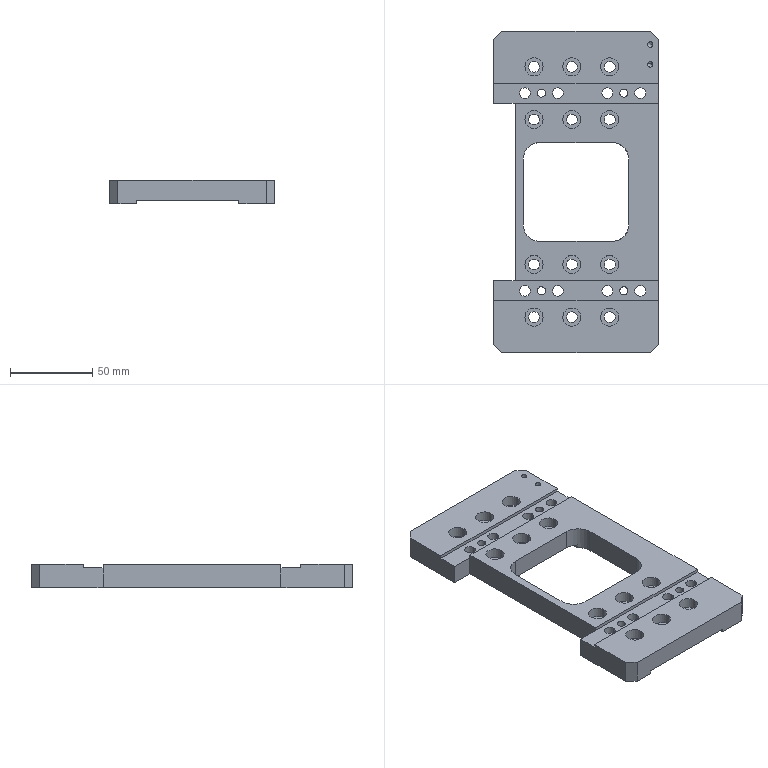Component | SolidWorks | 17081801-804-001A-1 | 1 solid | 155 faces | box 100 x 195 x 14 mm | volume 162308 mm3 | cylinder 96 | plane 55 | cone 4 | commonest cylinder face diameters 11 x40 6.6 x40 5 x8 3.3 x4 20 x4 | material AL6061
build123d program:
from build123d import *

# Parameters (mm, degrees)
SKETCH1_W                                       = 195
SKETCH1_H                                       = 100
BOSS_EXTRUDE1_DEPTH                             = 7
M6_HEX_SOCKET_HEAD_CAP_SCREW_CBORE1_D           = 6.6
M6_HEX_SOCKET_HEAD_CAP_SCREW_CBORE1_CBORE_D     = 11
M6_HEX_SOCKET_HEAD_CAP_SCREW_CBORE1_CBORE_DEPTH = 6.4
LPATTERN1_COUNT                                 = 2
LPATTERN1_PITCH                                 = 120
M6_HEX_SOCKET_HEAD_CAP_SCREW_CBORE2_D           = 6.6
M6_HEX_SOCKET_HEAD_CAP_SCREW_CBORE2_DEPTH       = 56
M6_HEX_SOCKET_HEAD_CAP_SCREW_CBORE2_CBORE_D     = 11
M6_HEX_SOCKET_HEAD_CAP_SCREW_CBORE2_CBORE_DEPTH = 6.4
M6_HEX_SOCKET_HEAD_CAP_SCREW_CBORE2_TIP         = 1.983
CHAMFER1_SIZE                                   = 5
SKETCH9_W                                       = 60
SKETCH9_H                                       = 64
CUT_EXTRUDE1_DEPTH                              = 111.464
FILLET1_R                                       = 10
M4_TAPPED_HOLE1_D                               = 3.3
M4_TAPPED_HOLE1_DEPTH                           = 10.1
M4_TAPPED_HOLE1_TIP                             = 0.9914
SKETCH12_W                                      = 195
SKETCH12_H                                      = 62
CUT_EXTRUDE2_DEPTH                              = 2
SKETCH13_W                                      = 12
SKETCH13_H                                      = 120
CUT_EXTRUDE3_DEPTH                              = 2
SIZE_MM_DOWEL_PIN_HOLE1_D                       = 5
SKETCH16_W                                      = 108
SKETCH16_H                                      = 13
CUT_EXTRUDE4_DEPTH                              = 111.464


with BuildPart() as part:
    # Sketch1 → Boss-Extrude1 (new, symmetric)
    with BuildSketch(Plane(origin=(0, 0, 0), x_dir=(1, 0, 0), z_dir=(0, 1, 0))):
        Rectangle(SKETCH1_W, SKETCH1_H)
    extrude(amount=BOSS_EXTRUDE1_DEPTH, both=True)

    # M6 Hex Socket Head Cap Screw CBORE1 (through all)
    with Locations(Plane(origin=(0, 7, 0), x_dir=(1, 0, 0), z_dir=(0, 1, 0))):
        with Locations((-76, 25.5), (-44, 25.5), (-44, -20.5), (-76, -20.5), (-76, 2.5), (-44, 2.5)):
            m6_hex_socket_head_cap_screw_cbore1 = CounterBoreHole(M6_HEX_SOCKET_HEAD_CAP_SCREW_CBORE1_D / 2, M6_HEX_SOCKET_HEAD_CAP_SCREW_CBORE1_CBORE_D / 2, M6_HEX_SOCKET_HEAD_CAP_SCREW_CBORE1_CBORE_DEPTH)

    # LPattern1: M6 Hex Socket Head Cap Screw CBORE1 ×2
    with Locations(*[(i * LPATTERN1_PITCH, 0, 0) for i in range(1, LPATTERN1_COUNT)]):
        add(m6_hex_socket_head_cap_screw_cbore1, mode=Mode.SUBTRACT)

    # M6 Hex Socket Head Cap Screw CBORE2
    with Locations(Plane.XZ.offset(7)):
        with Locations((60, -11), (60, 19), (60, 39), (-60, -11), (-60, 19), (-60, 39), (60, -31), (-60, -31)):
            CounterBoreHole(M6_HEX_SOCKET_HEAD_CAP_SCREW_CBORE2_D / 2, M6_HEX_SOCKET_HEAD_CAP_SCREW_CBORE2_CBORE_D / 2, M6_HEX_SOCKET_HEAD_CAP_SCREW_CBORE2_CBORE_DEPTH, depth=M6_HEX_SOCKET_HEAD_CAP_SCREW_CBORE2_DEPTH)
            with Locations((0, 0, -(M6_HEX_SOCKET_HEAD_CAP_SCREW_CBORE2_DEPTH + M6_HEX_SOCKET_HEAD_CAP_SCREW_CBORE2_TIP / 2))):  # 118° drill point
                Cone(0, M6_HEX_SOCKET_HEAD_CAP_SCREW_CBORE2_D / 2, M6_HEX_SOCKET_HEAD_CAP_SCREW_CBORE2_TIP, mode=Mode.SUBTRACT)

    # Chamfer1
    chamfer1_edges = [part.edges().sort_by_distance(p)[0] for p in [
        (-97.5, 0, -50),
        (97.5, 0, -50),
        (97.5, 0, 50),
        (-97.5, 0, 50),
    ]]
    chamfer(chamfer1_edges, length=CHAMFER1_SIZE)

    # Sketch9 → Cut-Extrude1 (cut, through all)
    with BuildSketch(Plane(origin=(0, 7, 0), x_dir=(1, 0, 0), z_dir=(0, 1, 0))):
        Rectangle(SKETCH9_W, SKETCH9_H)
    extrude(amount=-CUT_EXTRUDE1_DEPTH, mode=Mode.SUBTRACT)

    # Fillet1
    fillet1_edges = [part.edges().sort_by_distance(p)[0] for p in [
        (-30, 0, 32),
        (-30, 0, -32),
        (30, 0, -32),
        (30, 0, 32),
    ]]
    fillet(fillet1_edges, radius=FILLET1_R)

    # M4 Tapped Hole1
    with Locations(Plane(origin=(0, 7, 0), x_dir=(-1, 0, 0), z_dir=(0, 1, 0))):
        with Locations((-77.5, 45), (-89.5, 45)):
            Hole(M4_TAPPED_HOLE1_D / 2, depth=M4_TAPPED_HOLE1_DEPTH)
            with Locations((0, 0, -(M4_TAPPED_HOLE1_DEPTH + M4_TAPPED_HOLE1_TIP / 2))):  # 118° drill point
                Cone(0, M4_TAPPED_HOLE1_D / 2, M4_TAPPED_HOLE1_TIP, mode=Mode.SUBTRACT)

    # Sketch12 → Cut-Extrude2 (cut)
    with BuildSketch(Plane.XZ.offset(7)):
        with Locations((0, -2.5)):
            Rectangle(SKETCH12_W, SKETCH12_H)
    extrude(amount=-CUT_EXTRUDE2_DEPTH, mode=Mode.SUBTRACT)

    # Sketch13 → Cut-Extrude3 (cut)
    with BuildSketch(Plane(origin=(0, 7, 0), x_dir=(1, 0, 0), z_dir=(0, 1, 0))):
        with Locations((60, 0)):
            Rectangle(SKETCH13_W, SKETCH13_H)
        with Locations((-60, 0)):
            Rectangle(SKETCH13_W, SKETCH13_H)
    extrude(amount=-CUT_EXTRUDE3_DEPTH, mode=Mode.SUBTRACT)

    # Size mm Dowel Pin Hole1 (through all)
    with Locations(Plane(origin=(0, 5, 0), x_dir=(1, 0, 0), z_dir=(0, 1, 0))):
        with Locations((-60, 21), (60, 21), (60, -29), (-60, -29)):
            Hole(SIZE_MM_DOWEL_PIN_HOLE1_D / 2)

    # Sketch16 → Cut-Extrude4 (cut, through all)
    with BuildSketch(Plane(origin=(0, 7, 0), x_dir=(1, 0, 0), z_dir=(0, 1, 0))):
        with Locations((0, 43.5)):
            Rectangle(SKETCH16_W, SKETCH16_H)
    extrude(amount=-CUT_EXTRUDE4_DEPTH, mode=Mode.SUBTRACT)


solid = part.part

# Placed as in the assembly
solid = solid.moved(Location((-18.5, 2034.4, 127), (90, 90, 0)))